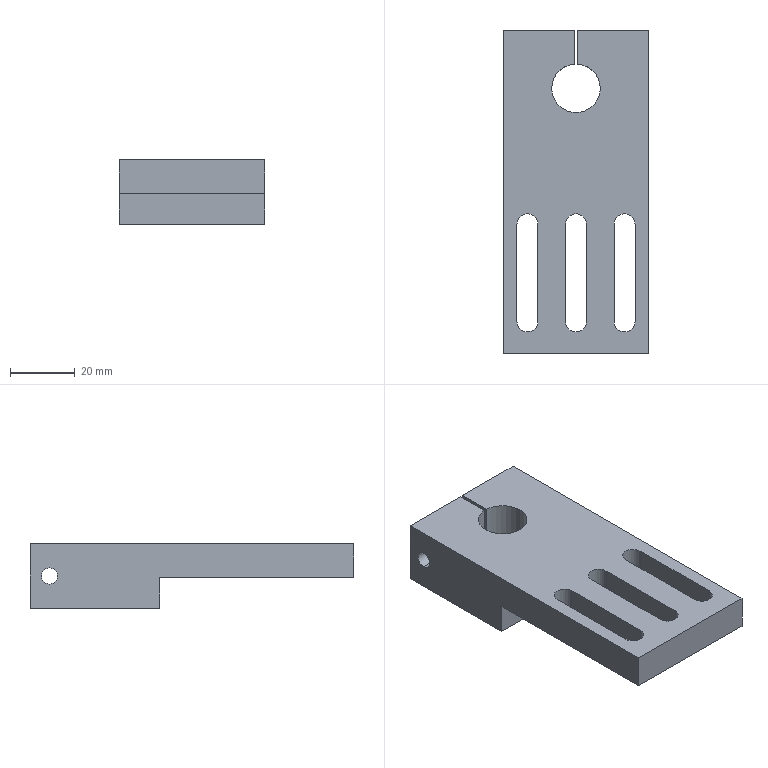Component | SolidWorks | DC-024-24-1 | 1 solid | 33 faces | box 45 x 100 x 20 mm | volume 51844 mm3 | plane 18 | cylinder 15 | commonest cylinder face diameters 6.5 x6 15 x3 5 x2 11 x2 6.6 x2
STEP:
#1=COLOUR_RGB('',0.7922,0.8196,0.9333);
#2=FILL_AREA_STYLE_COLOUR('',#1);
#3=FILL_AREA_STYLE('',(#2));
#4=SURFACE_STYLE_FILL_AREA(#3);
#5=SURFACE_SIDE_STYLE('',(#4));
#6=SURFACE_STYLE_USAGE(.BOTH.,#5);
#7=PRESENTATION_STYLE_ASSIGNMENT((#6));
#8=CARTESIAN_POINT('',(-1.895,12.89,0.6299));
#9=VERTEX_POINT('',#8);
#10=CARTESIAN_POINT('',(-1.895,12.89,0.4331));
#11=VERTEX_POINT('',#10);
#12=CARTESIAN_POINT('',(-1.895,12.89,0.5315));
#13=DIRECTION('',(1.,0.,0.));
#14=DIRECTION('',(0.,0.,-1.));
#15=AXIS2_PLACEMENT_3D('',#12,#13,#14);
#16=CIRCLE('',#15,0.09843);
#17=EDGE_CURVE('',#9,#11,#16,.T.);
#18=ORIENTED_EDGE('',*,*,#17,.F.);
#19=CARTESIAN_POINT('',(-1.029,12.89,0.6299));
#20=VERTEX_POINT('',#19);
#21=CARTESIAN_POINT('',(-1.029,12.89,0.6299));
#22=DIRECTION('',(1.,0.,0.));
#23=VECTOR('',#22,39.37);
#24=LINE('',#21,#23);
#25=EDGE_CURVE('',#9,#20,#24,.T.);
#26=ORIENTED_EDGE('',*,*,#25,.T.);
#27=CARTESIAN_POINT('',(-1.029,12.89,0.4331));
#28=VERTEX_POINT('',#27);
#29=CARTESIAN_POINT('',(-1.029,12.89,0.5315));
#30=DIRECTION('',(1.,0.,0.));
#31=DIRECTION('',(0.,0.,-1.));
#32=AXIS2_PLACEMENT_3D('',#29,#30,#31);
#33=CIRCLE('',#32,0.09843);
#34=EDGE_CURVE('',#20,#28,#33,.T.);
#35=ORIENTED_EDGE('',*,*,#34,.T.);
#36=CARTESIAN_POINT('',(-1.029,12.89,0.4331));
#37=DIRECTION('',(1.,0.,0.));
#38=VECTOR('',#37,39.37);
#39=LINE('',#36,#38);
#40=EDGE_CURVE('',#11,#28,#39,.T.);
#41=ORIENTED_EDGE('',*,*,#40,.F.);
#42=EDGE_LOOP('',(#18,#26,#35,#41));
#43=FACE_OUTER_BOUND('',#42,.T.);
#44=CARTESIAN_POINT('',(-1.029,12.89,0.5315));
#45=DIRECTION('',(1.,0.,0.));
#46=DIRECTION('',(0.,0.,-1.));
#47=AXIS2_PLACEMENT_3D('',#44,#45,#46);
#48=CYLINDRICAL_SURFACE('',#47,0.09843);
#49=ADVANCED_FACE('',(#43),#48,.F.);
#50=CARTESIAN_POINT('',(-0.3753,12.89,0.748));
#51=VERTEX_POINT('',#50);
#52=CARTESIAN_POINT('',(-0.3753,12.89,0.315));
#53=VERTEX_POINT('',#52);
#54=CARTESIAN_POINT('',(-0.3753,12.89,0.5315));
#55=DIRECTION('',(1.,0.,0.));
#56=DIRECTION('',(0.,0.,-1.));
#57=AXIS2_PLACEMENT_3D('',#54,#55,#56);
#58=CIRCLE('',#57,0.2165);
#59=EDGE_CURVE('',#51,#53,#58,.T.);
#60=ORIENTED_EDGE('',*,*,#59,.F.);
#61=CARTESIAN_POINT('',(-0.1233,12.89,0.748));
#62=VERTEX_POINT('',#61);
#63=CARTESIAN_POINT('',(-0.1233,12.89,0.748));
#64=DIRECTION('',(1.,0.,0.));
#65=VECTOR('',#64,39.37);
#66=LINE('',#63,#65);
#67=EDGE_CURVE('',#51,#62,#66,.T.);
#68=ORIENTED_EDGE('',*,*,#67,.T.);
#69=CARTESIAN_POINT('',(-0.1233,12.89,0.315));
#70=VERTEX_POINT('',#69);
#71=CARTESIAN_POINT('',(-0.1233,12.89,0.5315));
#72=DIRECTION('',(1.,0.,0.));
#73=DIRECTION('',(0.,0.,-1.));
#74=AXIS2_PLACEMENT_3D('',#71,#72,#73);
#75=CIRCLE('',#74,0.2165);
#76=EDGE_CURVE('',#62,#70,#75,.T.);
#77=ORIENTED_EDGE('',*,*,#76,.T.);
#78=CARTESIAN_POINT('',(-0.1233,12.89,0.315));
#79=DIRECTION('',(1.,0.,0.));
#80=VECTOR('',#79,39.37);
#81=LINE('',#78,#80);
#82=EDGE_CURVE('',#53,#70,#81,.T.);
#83=ORIENTED_EDGE('',*,*,#82,.F.);
#84=EDGE_LOOP('',(#60,#68,#77,#83));
#85=FACE_OUTER_BOUND('',#84,.T.);
#86=CARTESIAN_POINT('',(-0.1233,12.89,0.5315));
#87=DIRECTION('',(1.,0.,0.));
#88=DIRECTION('',(0.,0.,-1.));
#89=AXIS2_PLACEMENT_3D('',#86,#87,#88);
#90=CYLINDRICAL_SURFACE('',#89,0.2165);
#91=ADVANCED_FACE('',(#85),#90,.F.);
#92=CARTESIAN_POINT('',(-0.9895,12.89,0.6614));
#93=VERTEX_POINT('',#92);
#94=CARTESIAN_POINT('',(-0.9895,12.89,0.4016));
#95=VERTEX_POINT('',#94);
#96=CARTESIAN_POINT('',(-0.9895,12.89,0.5315));
#97=DIRECTION('',(1.,0.,0.));
#98=DIRECTION('',(0.,0.,-1.));
#99=AXIS2_PLACEMENT_3D('',#96,#97,#98);
#100=CIRCLE('',#99,0.1299);
#101=EDGE_CURVE('',#93,#95,#100,.T.);
#102=ORIENTED_EDGE('',*,*,#101,.F.);
#103=CARTESIAN_POINT('',(-0.3753,12.89,0.6614));
#104=VERTEX_POINT('',#103);
#105=CARTESIAN_POINT('',(-0.1233,12.89,0.6614));
#106=DIRECTION('',(1.,0.,0.));
#107=VECTOR('',#106,39.37);
#108=LINE('',#105,#107);
#109=EDGE_CURVE('',#93,#104,#108,.T.);
#110=ORIENTED_EDGE('',*,*,#109,.T.);
#111=CARTESIAN_POINT('',(-0.3753,12.89,0.4016));
#112=VERTEX_POINT('',#111);
#113=CARTESIAN_POINT('',(-0.3753,12.89,0.5315));
#114=DIRECTION('',(1.,0.,0.));
#115=DIRECTION('',(0.,0.,-1.));
#116=AXIS2_PLACEMENT_3D('',#113,#114,#115);
#117=CIRCLE('',#116,0.1299);
#118=EDGE_CURVE('',#104,#112,#117,.T.);
#119=ORIENTED_EDGE('',*,*,#118,.T.);
#120=CARTESIAN_POINT('',(-0.1233,12.89,0.4016));
#121=DIRECTION('',(1.,0.,0.));
#122=VECTOR('',#121,39.37);
#123=LINE('',#120,#122);
#124=EDGE_CURVE('',#95,#112,#123,.T.);
#125=ORIENTED_EDGE('',*,*,#124,.F.);
#126=EDGE_LOOP('',(#102,#110,#119,#125));
#127=FACE_OUTER_BOUND('',#126,.T.);
#128=CARTESIAN_POINT('',(-0.1233,12.89,0.5315));
#129=DIRECTION('',(1.,0.,0.));
#130=DIRECTION('',(0.,0.,-1.));
#131=AXIS2_PLACEMENT_3D('',#128,#129,#130);
#132=CYLINDRICAL_SURFACE('',#131,0.1299);
#133=ADVANCED_FACE('',(#127),#132,.F.);
#134=CARTESIAN_POINT('',(-0.7139,12.418,0.1378));
#135=VERTEX_POINT('',#134);
#136=CARTESIAN_POINT('',(-1.304,12.418,0.1378));
#137=VERTEX_POINT('',#136);
#138=CARTESIAN_POINT('',(-1.009,12.418,0.1378));
#139=DIRECTION('',(0.,0.,-1.));
#140=DIRECTION('',(1.,0.,0.));
#141=AXIS2_PLACEMENT_3D('',#138,#139,#140);
#142=CIRCLE('',#141,0.2953);
#143=EDGE_CURVE('',#135,#137,#142,.T.);
#144=ORIENTED_EDGE('',*,*,#143,.T.);
#145=CARTESIAN_POINT('',(-1.304,12.418,0.9252));
#146=VERTEX_POINT('',#145);
#147=CARTESIAN_POINT('',(-1.304,12.418,-0.6974));
#148=DIRECTION('',(0.,0.,1.));
#149=VECTOR('',#148,39.37);
#150=LINE('',#147,#149);
#151=EDGE_CURVE('',#137,#146,#150,.T.);
#152=ORIENTED_EDGE('',*,*,#151,.T.);
#153=CARTESIAN_POINT('',(-0.7139,12.418,0.9252));
#154=VERTEX_POINT('',#153);
#155=CARTESIAN_POINT('',(-1.009,12.418,0.9252));
#156=DIRECTION('',(0.,0.,1.));
#157=DIRECTION('',(1.,0.,0.));
#158=AXIS2_PLACEMENT_3D('',#155,#156,#157);
#159=CIRCLE('',#158,0.2953);
#160=EDGE_CURVE('',#146,#154,#159,.T.);
#161=ORIENTED_EDGE('',*,*,#160,.T.);
#162=CARTESIAN_POINT('',(-0.7139,12.418,-0.6974));
#163=DIRECTION('',(0.,0.,1.));
#164=VECTOR('',#163,39.37);
#165=LINE('',#162,#164);
#166=EDGE_CURVE('',#135,#154,#165,.T.);
#167=ORIENTED_EDGE('',*,*,#166,.F.);
#168=EDGE_LOOP('',(#144,#152,#161,#167));
#169=FACE_OUTER_BOUND('',#168,.T.);
#170=CARTESIAN_POINT('',(-1.009,12.418,-0.6974));
#171=DIRECTION('',(0.,0.,1.));
#172=DIRECTION('',(1.,0.,0.));
#173=AXIS2_PLACEMENT_3D('',#170,#171,#172);
#174=CYLINDRICAL_SURFACE('',#173,0.2953);
#175=ADVANCED_FACE('',(#169),#174,.F.);
#176=CARTESIAN_POINT('',(-0.9895,12.712,0.1378));
#177=VERTEX_POINT('',#176);
#178=CARTESIAN_POINT('',(-1.009,12.418,0.1378));
#179=DIRECTION('',(0.,0.,-1.));
#180=DIRECTION('',(1.,0.,0.));
#181=AXIS2_PLACEMENT_3D('',#178,#179,#180);
#182=CIRCLE('',#181,0.2953);
#183=EDGE_CURVE('',#177,#135,#182,.T.);
#184=ORIENTED_EDGE('',*,*,#183,.T.);
#185=ORIENTED_EDGE('',*,*,#166,.T.);
#186=CARTESIAN_POINT('',(-0.9895,12.712,0.9252));
#187=VERTEX_POINT('',#186);
#188=CARTESIAN_POINT('',(-1.009,12.418,0.9252));
#189=DIRECTION('',(0.,0.,1.));
#190=DIRECTION('',(1.,0.,0.));
#191=AXIS2_PLACEMENT_3D('',#188,#189,#190);
#192=CIRCLE('',#191,0.2953);
#193=EDGE_CURVE('',#154,#187,#192,.T.);
#194=ORIENTED_EDGE('',*,*,#193,.T.);
#195=CARTESIAN_POINT('',(-0.9895,12.712,-0.6974));
#196=DIRECTION('',(0.,0.,-1.));
#197=VECTOR('',#196,39.37);
#198=LINE('',#195,#197);
#199=EDGE_CURVE('',#187,#177,#198,.T.);
#200=ORIENTED_EDGE('',*,*,#199,.T.);
#201=EDGE_LOOP('',(#184,#185,#194,#200));
#202=FACE_OUTER_BOUND('',#201,.T.);
#203=CARTESIAN_POINT('',(-1.009,12.418,-0.6974));
#204=DIRECTION('',(0.,0.,1.));
#205=DIRECTION('',(1.,0.,0.));
#206=AXIS2_PLACEMENT_3D('',#203,#204,#205);
#207=CYLINDRICAL_SURFACE('',#206,0.2953);
#208=ADVANCED_FACE('',(#202),#207,.F.);
#209=CARTESIAN_POINT('',(-0.1233,9.189,0.9252));
#210=VERTEX_POINT('',#209);
#211=CARTESIAN_POINT('',(-0.1233,9.189,0.5118));
#212=VERTEX_POINT('',#211);
#213=CARTESIAN_POINT('',(-0.1233,9.189,0.9252));
#214=DIRECTION('',(0.,0.,-1.));
#215=VECTOR('',#214,39.37);
#216=LINE('',#213,#215);
#217=EDGE_CURVE('',#210,#212,#216,.T.);
#218=ORIENTED_EDGE('',*,*,#217,.T.);
#219=CARTESIAN_POINT('',(-0.1233,11.552,0.5118));
#220=VERTEX_POINT('',#219);
#221=CARTESIAN_POINT('',(-0.1233,9.189,0.5118));
#222=DIRECTION('',(0.,-1.,0.));
#223=VECTOR('',#222,39.37);
#224=LINE('',#221,#223);
#225=EDGE_CURVE('',#220,#212,#224,.T.);
#226=ORIENTED_EDGE('',*,*,#225,.F.);
#227=CARTESIAN_POINT('',(-0.1233,11.552,0.1378));
#228=VERTEX_POINT('',#227);
#229=CARTESIAN_POINT('',(-0.1233,11.552,0.1378));
#230=DIRECTION('',(0.,-0.,1.));
#231=VECTOR('',#230,39.37);
#232=LINE('',#229,#231);
#233=EDGE_CURVE('',#228,#220,#232,.T.);
#234=ORIENTED_EDGE('',*,*,#233,.F.);
#235=CARTESIAN_POINT('',(-0.1233,13.126,0.1378));
#236=VERTEX_POINT('',#235);
#237=CARTESIAN_POINT('',(-0.1233,9.189,0.1378));
#238=DIRECTION('',(0.,1.,0.));
#239=VECTOR('',#238,39.37);
#240=LINE('',#237,#239);
#241=EDGE_CURVE('',#228,#236,#240,.T.);
#242=ORIENTED_EDGE('',*,*,#241,.T.);
#243=CARTESIAN_POINT('',(-0.1233,13.126,0.9252));
#244=VERTEX_POINT('',#243);
#245=CARTESIAN_POINT('',(-0.1233,13.126,0.9252));
#246=DIRECTION('',(0.,0.,-1.));
#247=VECTOR('',#246,39.37);
#248=LINE('',#245,#247);
#249=EDGE_CURVE('',#244,#236,#248,.T.);
#250=ORIENTED_EDGE('',*,*,#249,.F.);
#251=CARTESIAN_POINT('',(-0.1233,9.189,0.9252));
#252=DIRECTION('',(0.,1.,0.));
#253=VECTOR('',#252,39.37);
#254=LINE('',#251,#253);
#255=EDGE_CURVE('',#210,#244,#254,.T.);
#256=ORIENTED_EDGE('',*,*,#255,.F.);
#257=EDGE_LOOP('',(#218,#226,#234,#242,#250,#256));
#258=FACE_OUTER_BOUND('',#257,.T.);
#259=CARTESIAN_POINT('',(-0.1233,12.89,0.5315));
#260=DIRECTION('',(1.,0.,0.));
#261=DIRECTION('',(0.,0.,-1.));
#262=AXIS2_PLACEMENT_3D('',#259,#260,#261);
#263=CIRCLE('',#262,0.2165);
#264=EDGE_CURVE('',#70,#62,#263,.T.);
#265=ORIENTED_EDGE('',*,*,#264,.F.);
#266=ORIENTED_EDGE('',*,*,#76,.F.);
#267=EDGE_LOOP('',(#265,#266));
#268=FACE_BOUND('',#267,.T.);
#269=CARTESIAN_POINT('',(-0.1233,9.189,0.9252));
#270=DIRECTION('',(-1.,0.,0.));
#271=DIRECTION('',(0.,0.,1.));
#272=AXIS2_PLACEMENT_3D('',#269,#270,#271);
#273=PLANE('',#272);
#274=ADVANCED_FACE('',(#258,#268),#273,.F.);
#275=CARTESIAN_POINT('',(-1.029,13.126,0.9252));
#276=VERTEX_POINT('',#275);
#277=CARTESIAN_POINT('',(-1.895,13.126,0.9252));
#278=VERTEX_POINT('',#277);
#279=CARTESIAN_POINT('',(-0.1233,13.126,0.9252));
#280=DIRECTION('',(-1.,-0.,0.));
#281=VECTOR('',#280,39.37);
#282=LINE('',#279,#281);
#283=EDGE_CURVE('',#276,#278,#282,.T.);
#284=ORIENTED_EDGE('',*,*,#283,.F.);
#285=CARTESIAN_POINT('',(-1.029,13.126,0.1378));
#286=VERTEX_POINT('',#285);
#287=CARTESIAN_POINT('',(-1.029,13.126,0.9252));
#288=DIRECTION('',(0.,0.,-1.));
#289=VECTOR('',#288,39.37);
#290=LINE('',#287,#289);
#291=EDGE_CURVE('',#276,#286,#290,.T.);
#292=ORIENTED_EDGE('',*,*,#291,.T.);
#293=CARTESIAN_POINT('',(-1.895,13.126,0.1378));
#294=VERTEX_POINT('',#293);
#295=CARTESIAN_POINT('',(-0.1233,13.126,0.1378));
#296=DIRECTION('',(-1.,-0.,0.));
#297=VECTOR('',#296,39.37);
#298=LINE('',#295,#297);
#299=EDGE_CURVE('',#286,#294,#298,.T.);
#300=ORIENTED_EDGE('',*,*,#299,.T.);
#301=CARTESIAN_POINT('',(-1.895,13.126,0.9252));
#302=DIRECTION('',(0.,0.,-1.));
#303=VECTOR('',#302,39.37);
#304=LINE('',#301,#303);
#305=EDGE_CURVE('',#278,#294,#304,.T.);
#306=ORIENTED_EDGE('',*,*,#305,.F.);
#307=EDGE_LOOP('',(#284,#292,#300,#306));
#308=FACE_OUTER_BOUND('',#307,.T.);
#309=CARTESIAN_POINT('',(-0.1233,13.126,0.9252));
#310=DIRECTION('',(0.,-1.,0.));
#311=DIRECTION('',(1.,0.,0.));
#312=AXIS2_PLACEMENT_3D('',#309,#310,#311);
#313=PLANE('',#312);
#314=ADVANCED_FACE('',(#308),#313,.F.);
#315=CARTESIAN_POINT('',(-1.895,12.89,0.5315));
#316=DIRECTION('',(1.,0.,0.));
#317=DIRECTION('',(0.,0.,-1.));
#318=AXIS2_PLACEMENT_3D('',#315,#316,#317);
#319=CIRCLE('',#318,0.09843);
#320=EDGE_CURVE('',#11,#9,#319,.T.);
#321=ORIENTED_EDGE('',*,*,#320,.T.);
#322=ORIENTED_EDGE('',*,*,#17,.T.);
#323=EDGE_LOOP('',(#321,#322));
#324=FACE_BOUND('',#323,.T.);
#325=CARTESIAN_POINT('',(-1.895,11.552,0.5118));
#326=VERTEX_POINT('',#325);
#327=CARTESIAN_POINT('',(-1.895,11.552,0.1378));
#328=VERTEX_POINT('',#327);
#329=CARTESIAN_POINT('',(-1.895,11.552,0.1378));
#330=DIRECTION('',(0.,0.,-1.));
#331=VECTOR('',#330,39.37);
#332=LINE('',#329,#331);
#333=EDGE_CURVE('',#326,#328,#332,.T.);
#334=ORIENTED_EDGE('',*,*,#333,.F.);
#335=CARTESIAN_POINT('',(-1.895,9.189,0.5118));
#336=VERTEX_POINT('',#335);
#337=CARTESIAN_POINT('',(-1.895,9.189,0.5118));
#338=DIRECTION('',(0.,1.,0.));
#339=VECTOR('',#338,39.37);
#340=LINE('',#337,#339);
#341=EDGE_CURVE('',#336,#326,#340,.T.);
#342=ORIENTED_EDGE('',*,*,#341,.F.);
#343=CARTESIAN_POINT('',(-1.895,9.189,0.9252));
#344=VERTEX_POINT('',#343);
#345=CARTESIAN_POINT('',(-1.895,9.189,0.9252));
#346=DIRECTION('',(0.,0.,-1.));
#347=VECTOR('',#346,39.37);
#348=LINE('',#345,#347);
#349=EDGE_CURVE('',#344,#336,#348,.T.);
#350=ORIENTED_EDGE('',*,*,#349,.F.);
#351=CARTESIAN_POINT('',(-1.895,9.189,0.9252));
#352=DIRECTION('',(0.,-1.,0.));
#353=VECTOR('',#352,39.37);
#354=LINE('',#351,#353);
#355=EDGE_CURVE('',#278,#344,#354,.T.);
#356=ORIENTED_EDGE('',*,*,#355,.F.);
#357=ORIENTED_EDGE('',*,*,#305,.T.);
#358=CARTESIAN_POINT('',(-1.895,9.189,0.1378));
#359=DIRECTION('',(0.,-1.,0.));
#360=VECTOR('',#359,39.37);
#361=LINE('',#358,#360);
#362=EDGE_CURVE('',#294,#328,#361,.T.);
#363=ORIENTED_EDGE('',*,*,#362,.T.);
#364=EDGE_LOOP('',(#334,#342,#350,#356,#357,#363));
#365=FACE_OUTER_BOUND('',#364,.T.);
#366=CARTESIAN_POINT('',(-1.895,9.189,0.9252));
#367=DIRECTION('',(1.,0.,0.));
#368=DIRECTION('',(0.,0.,-1.));
#369=AXIS2_PLACEMENT_3D('',#366,#367,#368);
#370=PLANE('',#369);
#371=ADVANCED_FACE('',(#324,#365),#370,.F.);
#372=ORIENTED_EDGE('',*,*,#349,.T.);
#373=CARTESIAN_POINT('',(-4.287,9.189,0.5118));
#374=DIRECTION('',(1.,0.,0.));
#375=VECTOR('',#374,39.37);
#376=LINE('',#373,#375);
#377=EDGE_CURVE('',#336,#212,#376,.T.);
#378=ORIENTED_EDGE('',*,*,#377,.T.);
#379=ORIENTED_EDGE('',*,*,#217,.F.);
#380=CARTESIAN_POINT('',(-0.1233,9.189,0.9252));
#381=DIRECTION('',(1.,0.,0.));
#382=VECTOR('',#381,39.37);
#383=LINE('',#380,#382);
#384=EDGE_CURVE('',#344,#210,#383,.T.);
#385=ORIENTED_EDGE('',*,*,#384,.F.);
#386=EDGE_LOOP('',(#372,#378,#379,#385));
#387=FACE_OUTER_BOUND('',#386,.T.);
#388=CARTESIAN_POINT('',(-0.1233,9.189,0.9252));
#389=DIRECTION('',(-0.,1.,0.));
#390=DIRECTION('',(-1.,-0.,0.));
#391=AXIS2_PLACEMENT_3D('',#388,#389,#390);
#392=PLANE('',#391);
#393=ADVANCED_FACE('',(#387),#392,.F.);
#394=CARTESIAN_POINT('',(-0.9895,13.126,0.1378));
#395=VERTEX_POINT('',#394);
#396=CARTESIAN_POINT('',(-0.1233,13.126,0.1378));
#397=DIRECTION('',(-1.,-0.,0.));
#398=VECTOR('',#397,39.37);
#399=LINE('',#396,#398);
#400=EDGE_CURVE('',#236,#395,#399,.T.);
#401=ORIENTED_EDGE('',*,*,#400,.T.);
#402=CARTESIAN_POINT('',(-0.9895,13.126,0.9252));
#403=VERTEX_POINT('',#402);
#404=CARTESIAN_POINT('',(-0.9895,13.126,0.9252));
#405=DIRECTION('',(0.,0.,1.));
#406=VECTOR('',#405,39.37);
#407=LINE('',#404,#406);
#408=EDGE_CURVE('',#395,#403,#407,.T.);
#409=ORIENTED_EDGE('',*,*,#408,.T.);
#410=CARTESIAN_POINT('',(-0.1233,13.126,0.9252));
#411=DIRECTION('',(-1.,-0.,0.));
#412=VECTOR('',#411,39.37);
#413=LINE('',#410,#412);
#414=EDGE_CURVE('',#244,#403,#413,.T.);
#415=ORIENTED_EDGE('',*,*,#414,.F.);
#416=ORIENTED_EDGE('',*,*,#249,.T.);
#417=EDGE_LOOP('',(#401,#409,#415,#416));
#418=FACE_OUTER_BOUND('',#417,.T.);
#419=CARTESIAN_POINT('',(-0.1233,13.126,0.9252));
#420=DIRECTION('',(0.,-1.,0.));
#421=DIRECTION('',(1.,0.,0.));
#422=AXIS2_PLACEMENT_3D('',#419,#420,#421);
#423=PLANE('',#422);
#424=ADVANCED_FACE('',(#418),#423,.F.);
#425=CARTESIAN_POINT('',(-1.472,10.764,0.9252));
#426=VERTEX_POINT('',#425);
#427=CARTESIAN_POINT('',(-1.728,10.764,0.9252));
#428=VERTEX_POINT('',#427);
#429=CARTESIAN_POINT('',(-1.6,10.764,0.9252));
#430=DIRECTION('',(0.,0.,1.));
#431=DIRECTION('',(1.,0.,0.));
#432=AXIS2_PLACEMENT_3D('',#429,#430,#431);
#433=CIRCLE('',#432,0.128);
#434=EDGE_CURVE('',#426,#428,#433,.T.);
#435=ORIENTED_EDGE('',*,*,#434,.F.);
#436=CARTESIAN_POINT('',(-1.472,9.583,0.9252));
#437=VERTEX_POINT('',#436);
#438=CARTESIAN_POINT('',(-1.472,10.764,0.9252));
#439=DIRECTION('',(-0.,1.,0.));
#440=VECTOR('',#439,39.37);
#441=LINE('',#438,#440);
#442=EDGE_CURVE('',#437,#426,#441,.T.);
#443=ORIENTED_EDGE('',*,*,#442,.F.);
#444=CARTESIAN_POINT('',(-1.728,9.583,0.9252));
#445=VERTEX_POINT('',#444);
#446=CARTESIAN_POINT('',(-1.6,9.583,0.9252));
#447=DIRECTION('',(0.,0.,1.));
#448=DIRECTION('',(1.,0.,0.));
#449=AXIS2_PLACEMENT_3D('',#446,#447,#448);
#450=CIRCLE('',#449,0.128);
#451=EDGE_CURVE('',#445,#437,#450,.T.);
#452=ORIENTED_EDGE('',*,*,#451,.F.);
#453=CARTESIAN_POINT('',(-1.728,10.764,0.9252));
#454=DIRECTION('',(0.,-1.,0.));
#455=VECTOR('',#454,39.37);
#456=LINE('',#453,#455);
#457=EDGE_CURVE('',#428,#445,#456,.T.);
#458=ORIENTED_EDGE('',*,*,#457,.F.);
#459=EDGE_LOOP('',(#435,#443,#452,#458));
#460=FACE_BOUND('',#459,.T.);
#461=CARTESIAN_POINT('',(-0.2907,10.764,0.9252));
#462=VERTEX_POINT('',#461);
#463=CARTESIAN_POINT('',(-0.5466,10.764,0.9252));
#464=VERTEX_POINT('',#463);
#465=CARTESIAN_POINT('',(-0.4186,10.764,0.9252));
#466=DIRECTION('',(0.,0.,1.));
#467=DIRECTION('',(1.,0.,0.));
#468=AXIS2_PLACEMENT_3D('',#465,#466,#467);
#469=CIRCLE('',#468,0.128);
#470=EDGE_CURVE('',#462,#464,#469,.T.);
#471=ORIENTED_EDGE('',*,*,#470,.F.);
#472=CARTESIAN_POINT('',(-0.2907,9.583,0.9252));
#473=VERTEX_POINT('',#472);
#474=CARTESIAN_POINT('',(-0.2907,10.764,0.9252));
#475=DIRECTION('',(-0.,1.,0.));
#476=VECTOR('',#475,39.37);
#477=LINE('',#474,#476);
#478=EDGE_CURVE('',#473,#462,#477,.T.);
#479=ORIENTED_EDGE('',*,*,#478,.F.);
#480=CARTESIAN_POINT('',(-0.5466,9.583,0.9252));
#481=VERTEX_POINT('',#480);
#482=CARTESIAN_POINT('',(-0.4186,9.583,0.9252));
#483=DIRECTION('',(0.,0.,1.));
#484=DIRECTION('',(1.,0.,0.));
#485=AXIS2_PLACEMENT_3D('',#482,#483,#484);
#486=CIRCLE('',#485,0.128);
#487=EDGE_CURVE('',#481,#473,#486,.T.);
#488=ORIENTED_EDGE('',*,*,#487,.F.);
#489=CARTESIAN_POINT('',(-0.5466,10.764,0.9252));
#490=DIRECTION('',(0.,-1.,0.));
#491=VECTOR('',#490,39.37);
#492=LINE('',#489,#491);
#493=EDGE_CURVE('',#464,#481,#492,.T.);
#494=ORIENTED_EDGE('',*,*,#493,.F.);
#495=EDGE_LOOP('',(#471,#479,#488,#494));
#496=FACE_BOUND('',#495,.T.);
#497=CARTESIAN_POINT('',(-0.8812,10.764,0.9252));
#498=VERTEX_POINT('',#497);
#499=CARTESIAN_POINT('',(-1.137,10.764,0.9252));
#500=VERTEX_POINT('',#499);
#501=CARTESIAN_POINT('',(-1.009,10.764,0.9252));
#502=DIRECTION('',(0.,0.,1.));
#503=DIRECTION('',(1.,0.,0.));
#504=AXIS2_PLACEMENT_3D('',#501,#502,#503);
#505=CIRCLE('',#504,0.128);
#506=EDGE_CURVE('',#498,#500,#505,.T.);
#507=ORIENTED_EDGE('',*,*,#506,.F.);
#508=CARTESIAN_POINT('',(-0.8812,9.583,0.9252));
#509=VERTEX_POINT('',#508);
#510=CARTESIAN_POINT('',(-0.8812,10.764,0.9252));
#511=DIRECTION('',(-0.,1.,0.));
#512=VECTOR('',#511,39.37);
#513=LINE('',#510,#512);
#514=EDGE_CURVE('',#509,#498,#513,.T.);
#515=ORIENTED_EDGE('',*,*,#514,.F.);
#516=CARTESIAN_POINT('',(-1.137,9.583,0.9252));
#517=VERTEX_POINT('',#516);
#518=CARTESIAN_POINT('',(-1.009,9.583,0.9252));
#519=DIRECTION('',(0.,0.,1.));
#520=DIRECTION('',(1.,0.,0.));
#521=AXIS2_PLACEMENT_3D('',#518,#519,#520);
#522=CIRCLE('',#521,0.128);
#523=EDGE_CURVE('',#517,#509,#522,.T.);
#524=ORIENTED_EDGE('',*,*,#523,.F.);
#525=CARTESIAN_POINT('',(-1.137,10.764,0.9252));
#526=DIRECTION('',(0.,-1.,0.));
#527=VECTOR('',#526,39.37);
#528=LINE('',#525,#527);
#529=EDGE_CURVE('',#500,#517,#528,.T.);
#530=ORIENTED_EDGE('',*,*,#529,.F.);
#531=EDGE_LOOP('',(#507,#515,#524,#530));
#532=FACE_BOUND('',#531,.T.);
#533=CARTESIAN_POINT('',(-1.029,12.712,0.9252));
#534=VERTEX_POINT('',#533);
#535=CARTESIAN_POINT('',(-1.029,14.13,0.9252));
#536=DIRECTION('',(0.,-1.,0.));
#537=VECTOR('',#536,39.37);
#538=LINE('',#535,#537);
#539=EDGE_CURVE('',#276,#534,#538,.T.);
#540=ORIENTED_EDGE('',*,*,#539,.F.);
#541=ORIENTED_EDGE('',*,*,#283,.T.);
#542=ORIENTED_EDGE('',*,*,#355,.T.);
#543=ORIENTED_EDGE('',*,*,#384,.T.);
#544=ORIENTED_EDGE('',*,*,#255,.T.);
#545=ORIENTED_EDGE('',*,*,#414,.T.);
#546=CARTESIAN_POINT('',(-0.9895,14.13,0.9252));
#547=DIRECTION('',(0.,1.,0.));
#548=VECTOR('',#547,39.37);
#549=LINE('',#546,#548);
#550=EDGE_CURVE('',#187,#403,#549,.T.);
#551=ORIENTED_EDGE('',*,*,#550,.F.);
#552=ORIENTED_EDGE('',*,*,#193,.F.);
#553=ORIENTED_EDGE('',*,*,#160,.F.);
#554=CARTESIAN_POINT('',(-1.009,12.418,0.9252));
#555=DIRECTION('',(0.,0.,1.));
#556=DIRECTION('',(1.,0.,0.));
#557=AXIS2_PLACEMENT_3D('',#554,#555,#556);
#558=CIRCLE('',#557,0.2953);
#559=EDGE_CURVE('',#534,#146,#558,.T.);
#560=ORIENTED_EDGE('',*,*,#559,.F.);
#561=EDGE_LOOP('',(#540,#541,#542,#543,#544,#545,#551,#552,#553,#560));
#562=FACE_OUTER_BOUND('',#561,.T.);
#563=CARTESIAN_POINT('',(-1.009,11.158,0.9252));
#564=DIRECTION('',(0.,0.,1.));
#565=DIRECTION('',(1.,0.,0.));
#566=AXIS2_PLACEMENT_3D('',#563,#564,#565);
#567=PLANE('',#566);
#568=ADVANCED_FACE('',(#460,#496,#532,#562),#567,.T.);
#569=ORIENTED_EDGE('',*,*,#241,.F.);
#570=CARTESIAN_POINT('',(-4.287,11.552,0.1378));
#571=DIRECTION('',(1.,0.,0.));
#572=VECTOR('',#571,39.37);
#573=LINE('',#570,#572);
#574=EDGE_CURVE('',#328,#228,#573,.T.);
#575=ORIENTED_EDGE('',*,*,#574,.F.);
#576=ORIENTED_EDGE('',*,*,#362,.F.);
#577=ORIENTED_EDGE('',*,*,#299,.F.);
#578=CARTESIAN_POINT('',(-1.029,12.712,0.1378));
#579=VERTEX_POINT('',#578);
#580=CARTESIAN_POINT('',(-1.029,14.13,0.1378));
#581=DIRECTION('',(0.,1.,0.));
#582=VECTOR('',#581,39.37);
#583=LINE('',#580,#582);
#584=EDGE_CURVE('',#579,#286,#583,.T.);
#585=ORIENTED_EDGE('',*,*,#584,.F.);
#586=CARTESIAN_POINT('',(-1.009,12.418,0.1378));
#587=DIRECTION('',(0.,0.,-1.));
#588=DIRECTION('',(1.,0.,0.));
#589=AXIS2_PLACEMENT_3D('',#586,#587,#588);
#590=CIRCLE('',#589,0.2953);
#591=EDGE_CURVE('',#137,#579,#590,.T.);
#592=ORIENTED_EDGE('',*,*,#591,.F.);
#593=ORIENTED_EDGE('',*,*,#143,.F.);
#594=ORIENTED_EDGE('',*,*,#183,.F.);
#595=CARTESIAN_POINT('',(-0.9895,14.13,0.1378));
#596=DIRECTION('',(0.,-1.,0.));
#597=VECTOR('',#596,39.37);
#598=LINE('',#595,#597);
#599=EDGE_CURVE('',#395,#177,#598,.T.);
#600=ORIENTED_EDGE('',*,*,#599,.F.);
#601=ORIENTED_EDGE('',*,*,#400,.F.);
#602=EDGE_LOOP('',(#569,#575,#576,#577,#585,#592,#593,#594,#600,#601));
#603=FACE_OUTER_BOUND('',#602,.T.);
#604=CARTESIAN_POINT('',(-1.009,11.158,0.1378));
#605=DIRECTION('',(0.,0.,1.));
#606=DIRECTION('',(1.,0.,0.));
#607=AXIS2_PLACEMENT_3D('',#604,#605,#606);
#608=PLANE('',#607);
#609=ADVANCED_FACE('',(#603),#608,.F.);
#610=ORIENTED_EDGE('',*,*,#151,.F.);
#611=ORIENTED_EDGE('',*,*,#591,.T.);
#612=CARTESIAN_POINT('',(-1.029,12.712,-0.6974));
#613=DIRECTION('',(0.,0.,1.));
#614=VECTOR('',#613,39.37);
#615=LINE('',#612,#614);
#616=EDGE_CURVE('',#579,#534,#615,.T.);
#617=ORIENTED_EDGE('',*,*,#616,.T.);
#618=ORIENTED_EDGE('',*,*,#559,.T.);
#619=EDGE_LOOP('',(#610,#611,#617,#618));
#620=FACE_OUTER_BOUND('',#619,.T.);
#621=CARTESIAN_POINT('',(-1.009,12.418,-0.6974));
#622=DIRECTION('',(0.,0.,1.));
#623=DIRECTION('',(1.,0.,0.));
#624=AXIS2_PLACEMENT_3D('',#621,#622,#623);
#625=CYLINDRICAL_SURFACE('',#624,0.2953);
#626=ADVANCED_FACE('',(#620),#625,.F.);
#627=CARTESIAN_POINT('',(-0.9895,12.89,0.5315));
#628=DIRECTION('',(1.,0.,0.));
#629=DIRECTION('',(0.,0.,-1.));
#630=AXIS2_PLACEMENT_3D('',#627,#628,#629);
#631=CIRCLE('',#630,0.1299);
#632=EDGE_CURVE('',#95,#93,#631,.T.);
#633=ORIENTED_EDGE('',*,*,#632,.T.);
#634=ORIENTED_EDGE('',*,*,#101,.T.);
#635=EDGE_LOOP('',(#633,#634));
#636=FACE_BOUND('',#635,.T.);
#637=ORIENTED_EDGE('',*,*,#599,.T.);
#638=ORIENTED_EDGE('',*,*,#199,.F.);
#639=ORIENTED_EDGE('',*,*,#550,.T.);
#640=ORIENTED_EDGE('',*,*,#408,.F.);
#641=EDGE_LOOP('',(#637,#638,#639,#640));
#642=FACE_OUTER_BOUND('',#641,.T.);
#643=CARTESIAN_POINT('',(-0.9895,14.13,-1.869));
#644=DIRECTION('',(1.,0.,0.));
#645=DIRECTION('',(0.,0.,-1.));
#646=AXIS2_PLACEMENT_3D('',#643,#644,#645);
#647=PLANE('',#646);
#648=ADVANCED_FACE('',(#636,#642),#647,.F.);
#649=CARTESIAN_POINT('',(-1.029,12.89,0.5315));
#650=DIRECTION('',(1.,0.,0.));
#651=DIRECTION('',(0.,0.,-1.));
#652=AXIS2_PLACEMENT_3D('',#649,#650,#651);
#653=CIRCLE('',#652,0.09843);
#654=EDGE_CURVE('',#28,#20,#653,.T.);
#655=ORIENTED_EDGE('',*,*,#654,.F.);
#656=ORIENTED_EDGE('',*,*,#34,.F.);
#657=EDGE_LOOP('',(#655,#656));
#658=FACE_BOUND('',#657,.T.);
#659=ORIENTED_EDGE('',*,*,#539,.T.);
#660=ORIENTED_EDGE('',*,*,#616,.F.);
#661=ORIENTED_EDGE('',*,*,#584,.T.);
#662=ORIENTED_EDGE('',*,*,#291,.F.);
#663=EDGE_LOOP('',(#659,#660,#661,#662));
#664=FACE_OUTER_BOUND('',#663,.T.);
#665=CARTESIAN_POINT('',(-1.029,14.13,-1.869));
#666=DIRECTION('',(-1.,0.,0.));
#667=DIRECTION('',(0.,0.,1.));
#668=AXIS2_PLACEMENT_3D('',#665,#666,#667);
#669=PLANE('',#668);
#670=ADVANCED_FACE('',(#658,#664),#669,.F.);
#671=ORIENTED_EDGE('',*,*,#109,.F.);
#672=ORIENTED_EDGE('',*,*,#632,.F.);
#673=ORIENTED_EDGE('',*,*,#124,.T.);
#674=CARTESIAN_POINT('',(-0.3753,12.89,0.5315));
#675=DIRECTION('',(1.,0.,0.));
#676=DIRECTION('',(0.,0.,-1.));
#677=AXIS2_PLACEMENT_3D('',#674,#675,#676);
#678=CIRCLE('',#677,0.1299);
#679=EDGE_CURVE('',#112,#104,#678,.T.);
#680=ORIENTED_EDGE('',*,*,#679,.T.);
#681=EDGE_LOOP('',(#671,#672,#673,#680));
#682=FACE_OUTER_BOUND('',#681,.T.);
#683=CARTESIAN_POINT('',(-0.1233,12.89,0.5315));
#684=DIRECTION('',(1.,0.,0.));
#685=DIRECTION('',(0.,0.,-1.));
#686=AXIS2_PLACEMENT_3D('',#683,#684,#685);
#687=CYLINDRICAL_SURFACE('',#686,0.1299);
#688=ADVANCED_FACE('',(#682),#687,.F.);
#689=ORIENTED_EDGE('',*,*,#679,.F.);
#690=ORIENTED_EDGE('',*,*,#118,.F.);
#691=EDGE_LOOP('',(#689,#690));
#692=FACE_BOUND('',#691,.T.);
#693=CARTESIAN_POINT('',(-0.3753,12.89,0.5315));
#694=DIRECTION('',(1.,0.,0.));
#695=DIRECTION('',(0.,0.,-1.));
#696=AXIS2_PLACEMENT_3D('',#693,#694,#695);
#697=CIRCLE('',#696,0.2165);
#698=EDGE_CURVE('',#53,#51,#697,.T.);
#699=ORIENTED_EDGE('',*,*,#698,.T.);
#700=ORIENTED_EDGE('',*,*,#59,.T.);
#701=EDGE_LOOP('',(#699,#700));
#702=FACE_OUTER_BOUND('',#701,.T.);
#703=CARTESIAN_POINT('',(-0.3753,13.02,0.5315));
#704=DIRECTION('',(-1.,0.,0.));
#705=DIRECTION('',(0.,0.,1.));
#706=AXIS2_PLACEMENT_3D('',#703,#704,#705);
#707=PLANE('',#706);
#708=ADVANCED_FACE('',(#692,#702),#707,.F.);
#709=ORIENTED_EDGE('',*,*,#67,.F.);
#710=ORIENTED_EDGE('',*,*,#698,.F.);
#711=ORIENTED_EDGE('',*,*,#82,.T.);
#712=ORIENTED_EDGE('',*,*,#264,.T.);
#713=EDGE_LOOP('',(#709,#710,#711,#712));
#714=FACE_OUTER_BOUND('',#713,.T.);
#715=CARTESIAN_POINT('',(-0.1233,12.89,0.5315));
#716=DIRECTION('',(1.,0.,0.));
#717=DIRECTION('',(0.,0.,-1.));
#718=AXIS2_PLACEMENT_3D('',#715,#716,#717);
#719=CYLINDRICAL_SURFACE('',#718,0.2165);
#720=ADVANCED_FACE('',(#714),#719,.F.);
#721=ORIENTED_EDGE('',*,*,#25,.F.);
#722=ORIENTED_EDGE('',*,*,#320,.F.);
#723=ORIENTED_EDGE('',*,*,#40,.T.);
#724=ORIENTED_EDGE('',*,*,#654,.T.);
#725=EDGE_LOOP('',(#721,#722,#723,#724));
#726=FACE_OUTER_BOUND('',#725,.T.);
#727=CARTESIAN_POINT('',(-1.029,12.89,0.5315));
#728=DIRECTION('',(1.,0.,0.));
#729=DIRECTION('',(0.,0.,-1.));
#730=AXIS2_PLACEMENT_3D('',#727,#728,#729);
#731=CYLINDRICAL_SURFACE('',#730,0.09843);
#732=ADVANCED_FACE('',(#726),#731,.F.);
#733=CARTESIAN_POINT('',(-1.137,10.764,0.5118));
#734=VERTEX_POINT('',#733);
#735=CARTESIAN_POINT('',(-1.137,10.764,-1.634));
#736=DIRECTION('',(0.,0.,1.));
#737=VECTOR('',#736,39.37);
#738=LINE('',#735,#737);
#739=EDGE_CURVE('',#734,#500,#738,.T.);
#740=ORIENTED_EDGE('',*,*,#739,.F.);
#741=CARTESIAN_POINT('',(-0.8812,10.764,0.5118));
#742=VERTEX_POINT('',#741);
#743=CARTESIAN_POINT('',(-1.009,10.764,0.5118));
#744=DIRECTION('',(0.,0.,-1.));
#745=DIRECTION('',(1.,0.,0.));
#746=AXIS2_PLACEMENT_3D('',#743,#744,#745);
#747=CIRCLE('',#746,0.128);
#748=EDGE_CURVE('',#734,#742,#747,.T.);
#749=ORIENTED_EDGE('',*,*,#748,.T.);
#750=CARTESIAN_POINT('',(-0.8812,10.764,-1.634));
#751=DIRECTION('',(0.,0.,1.));
#752=VECTOR('',#751,39.37);
#753=LINE('',#750,#752);
#754=EDGE_CURVE('',#742,#498,#753,.T.);
#755=ORIENTED_EDGE('',*,*,#754,.T.);
#756=ORIENTED_EDGE('',*,*,#506,.T.);
#757=EDGE_LOOP('',(#740,#749,#755,#756));
#758=FACE_OUTER_BOUND('',#757,.T.);
#759=CARTESIAN_POINT('',(-1.009,10.764,-1.634));
#760=DIRECTION('',(0.,0.,1.));
#761=DIRECTION('',(1.,0.,0.));
#762=AXIS2_PLACEMENT_3D('',#759,#760,#761);
#763=CYLINDRICAL_SURFACE('',#762,0.128);
#764=ADVANCED_FACE('',(#758),#763,.F.);
#765=ORIENTED_EDGE('',*,*,#754,.F.);
#766=CARTESIAN_POINT('',(-0.8812,9.583,0.5118));
#767=VERTEX_POINT('',#766);
#768=CARTESIAN_POINT('',(-0.8812,10.764,0.5118));
#769=DIRECTION('',(0.,-1.,0.));
#770=VECTOR('',#769,39.37);
#771=LINE('',#768,#770);
#772=EDGE_CURVE('',#742,#767,#771,.T.);
#773=ORIENTED_EDGE('',*,*,#772,.T.);
#774=CARTESIAN_POINT('',(-0.8812,9.583,-1.634));
#775=DIRECTION('',(0.,0.,1.));
#776=VECTOR('',#775,39.37);
#777=LINE('',#774,#776);
#778=EDGE_CURVE('',#767,#509,#777,.T.);
#779=ORIENTED_EDGE('',*,*,#778,.T.);
#780=ORIENTED_EDGE('',*,*,#514,.T.);
#781=EDGE_LOOP('',(#765,#773,#779,#780));
#782=FACE_OUTER_BOUND('',#781,.T.);
#783=CARTESIAN_POINT('',(-0.8812,10.764,-1.634));
#784=DIRECTION('',(1.,0.,0.));
#785=DIRECTION('',(-0.,1.,0.));
#786=AXIS2_PLACEMENT_3D('',#783,#784,#785);
#787=PLANE('',#786);
#788=ADVANCED_FACE('',(#782),#787,.F.);
#789=ORIENTED_EDGE('',*,*,#778,.F.);
#790=CARTESIAN_POINT('',(-1.137,9.583,0.5118));
#791=VERTEX_POINT('',#790);
#792=CARTESIAN_POINT('',(-1.009,9.583,0.5118));
#793=DIRECTION('',(0.,0.,-1.));
#794=DIRECTION('',(1.,0.,0.));
#795=AXIS2_PLACEMENT_3D('',#792,#793,#794);
#796=CIRCLE('',#795,0.128);
#797=EDGE_CURVE('',#767,#791,#796,.T.);
#798=ORIENTED_EDGE('',*,*,#797,.T.);
#799=CARTESIAN_POINT('',(-1.137,9.583,-1.634));
#800=DIRECTION('',(0.,0.,1.));
#801=VECTOR('',#800,39.37);
#802=LINE('',#799,#801);
#803=EDGE_CURVE('',#791,#517,#802,.T.);
#804=ORIENTED_EDGE('',*,*,#803,.T.);
#805=ORIENTED_EDGE('',*,*,#523,.T.);
#806=EDGE_LOOP('',(#789,#798,#804,#805));
#807=FACE_OUTER_BOUND('',#806,.T.);
#808=CARTESIAN_POINT('',(-1.009,9.583,-1.634));
#809=DIRECTION('',(0.,0.,1.));
#810=DIRECTION('',(1.,0.,0.));
#811=AXIS2_PLACEMENT_3D('',#808,#809,#810);
#812=CYLINDRICAL_SURFACE('',#811,0.128);
#813=ADVANCED_FACE('',(#807),#812,.F.);
#814=ORIENTED_EDGE('',*,*,#803,.F.);
#815=CARTESIAN_POINT('',(-1.137,10.764,0.5118));
#816=DIRECTION('',(-0.,1.,0.));
#817=VECTOR('',#816,39.37);
#818=LINE('',#815,#817);
#819=EDGE_CURVE('',#791,#734,#818,.T.);
#820=ORIENTED_EDGE('',*,*,#819,.T.);
#821=ORIENTED_EDGE('',*,*,#739,.T.);
#822=ORIENTED_EDGE('',*,*,#529,.T.);
#823=EDGE_LOOP('',(#814,#820,#821,#822));
#824=FACE_OUTER_BOUND('',#823,.T.);
#825=CARTESIAN_POINT('',(-1.137,10.764,-1.634));
#826=DIRECTION('',(-1.,-0.,0.));
#827=DIRECTION('',(0.,-1.,0.));
#828=AXIS2_PLACEMENT_3D('',#825,#826,#827);
#829=PLANE('',#828);
#830=ADVANCED_FACE('',(#824),#829,.F.);
#831=CARTESIAN_POINT('',(-0.5466,10.764,0.5118));
#832=VERTEX_POINT('',#831);
#833=CARTESIAN_POINT('',(-0.5466,10.764,-1.634));
#834=DIRECTION('',(0.,0.,1.));
#835=VECTOR('',#834,39.37);
#836=LINE('',#833,#835);
#837=EDGE_CURVE('',#832,#464,#836,.T.);
#838=ORIENTED_EDGE('',*,*,#837,.F.);
#839=CARTESIAN_POINT('',(-0.2907,10.764,0.5118));
#840=VERTEX_POINT('',#839);
#841=CARTESIAN_POINT('',(-0.4186,10.764,0.5118));
#842=DIRECTION('',(0.,0.,-1.));
#843=DIRECTION('',(1.,0.,0.));
#844=AXIS2_PLACEMENT_3D('',#841,#842,#843);
#845=CIRCLE('',#844,0.128);
#846=EDGE_CURVE('',#832,#840,#845,.T.);
#847=ORIENTED_EDGE('',*,*,#846,.T.);
#848=CARTESIAN_POINT('',(-0.2907,10.764,-1.634));
#849=DIRECTION('',(0.,0.,1.));
#850=VECTOR('',#849,39.37);
#851=LINE('',#848,#850);
#852=EDGE_CURVE('',#840,#462,#851,.T.);
#853=ORIENTED_EDGE('',*,*,#852,.T.);
#854=ORIENTED_EDGE('',*,*,#470,.T.);
#855=EDGE_LOOP('',(#838,#847,#853,#854));
#856=FACE_OUTER_BOUND('',#855,.T.);
#857=CARTESIAN_POINT('',(-0.4186,10.764,-1.634));
#858=DIRECTION('',(0.,0.,1.));
#859=DIRECTION('',(1.,0.,0.));
#860=AXIS2_PLACEMENT_3D('',#857,#858,#859);
#861=CYLINDRICAL_SURFACE('',#860,0.128);
#862=ADVANCED_FACE('',(#856),#861,.F.);
#863=ORIENTED_EDGE('',*,*,#852,.F.);
#864=CARTESIAN_POINT('',(-0.2907,9.583,0.5118));
#865=VERTEX_POINT('',#864);
#866=CARTESIAN_POINT('',(-0.2907,10.764,0.5118));
#867=DIRECTION('',(0.,-1.,0.));
#868=VECTOR('',#867,39.37);
#869=LINE('',#866,#868);
#870=EDGE_CURVE('',#840,#865,#869,.T.);
#871=ORIENTED_EDGE('',*,*,#870,.T.);
#872=CARTESIAN_POINT('',(-0.2907,9.583,-1.634));
#873=DIRECTION('',(0.,0.,1.));
#874=VECTOR('',#873,39.37);
#875=LINE('',#872,#874);
#876=EDGE_CURVE('',#865,#473,#875,.T.);
#877=ORIENTED_EDGE('',*,*,#876,.T.);
#878=ORIENTED_EDGE('',*,*,#478,.T.);
#879=EDGE_LOOP('',(#863,#871,#877,#878));
#880=FACE_OUTER_BOUND('',#879,.T.);
#881=CARTESIAN_POINT('',(-0.2907,10.764,-1.634));
#882=DIRECTION('',(1.,0.,0.));
#883=DIRECTION('',(-0.,1.,0.));
#884=AXIS2_PLACEMENT_3D('',#881,#882,#883);
#885=PLANE('',#884);
#886=ADVANCED_FACE('',(#880),#885,.F.);
#887=ORIENTED_EDGE('',*,*,#876,.F.);
#888=CARTESIAN_POINT('',(-0.5466,9.583,0.5118));
#889=VERTEX_POINT('',#888);
#890=CARTESIAN_POINT('',(-0.4186,9.583,0.5118));
#891=DIRECTION('',(0.,0.,-1.));
#892=DIRECTION('',(1.,0.,0.));
#893=AXIS2_PLACEMENT_3D('',#890,#891,#892);
#894=CIRCLE('',#893,0.128);
#895=EDGE_CURVE('',#865,#889,#894,.T.);
#896=ORIENTED_EDGE('',*,*,#895,.T.);
#897=CARTESIAN_POINT('',(-0.5466,9.583,-1.634));
#898=DIRECTION('',(0.,0.,1.));
#899=VECTOR('',#898,39.37);
#900=LINE('',#897,#899);
#901=EDGE_CURVE('',#889,#481,#900,.T.);
#902=ORIENTED_EDGE('',*,*,#901,.T.);
#903=ORIENTED_EDGE('',*,*,#487,.T.);
#904=EDGE_LOOP('',(#887,#896,#902,#903));
#905=FACE_OUTER_BOUND('',#904,.T.);
#906=CARTESIAN_POINT('',(-0.4186,9.583,-1.634));
#907=DIRECTION('',(0.,0.,1.));
#908=DIRECTION('',(1.,0.,0.));
#909=AXIS2_PLACEMENT_3D('',#906,#907,#908);
#910=CYLINDRICAL_SURFACE('',#909,0.128);
#911=ADVANCED_FACE('',(#905),#910,.F.);
#912=ORIENTED_EDGE('',*,*,#901,.F.);
#913=CARTESIAN_POINT('',(-0.5466,10.764,0.5118));
#914=DIRECTION('',(-0.,1.,0.));
#915=VECTOR('',#914,39.37);
#916=LINE('',#913,#915);
#917=EDGE_CURVE('',#889,#832,#916,.T.);
#918=ORIENTED_EDGE('',*,*,#917,.T.);
#919=ORIENTED_EDGE('',*,*,#837,.T.);
#920=ORIENTED_EDGE('',*,*,#493,.T.);
#921=EDGE_LOOP('',(#912,#918,#919,#920));
#922=FACE_OUTER_BOUND('',#921,.T.);
#923=CARTESIAN_POINT('',(-0.5466,10.764,-1.634));
#924=DIRECTION('',(-1.,-0.,0.));
#925=DIRECTION('',(0.,-1.,0.));
#926=AXIS2_PLACEMENT_3D('',#923,#924,#925);
#927=PLANE('',#926);
#928=ADVANCED_FACE('',(#922),#927,.F.);
#929=CARTESIAN_POINT('',(-1.728,10.764,0.5118));
#930=VERTEX_POINT('',#929);
#931=CARTESIAN_POINT('',(-1.728,10.764,-1.634));
#932=DIRECTION('',(0.,0.,1.));
#933=VECTOR('',#932,39.37);
#934=LINE('',#931,#933);
#935=EDGE_CURVE('',#930,#428,#934,.T.);
#936=ORIENTED_EDGE('',*,*,#935,.F.);
#937=CARTESIAN_POINT('',(-1.472,10.764,0.5118));
#938=VERTEX_POINT('',#937);
#939=CARTESIAN_POINT('',(-1.6,10.764,0.5118));
#940=DIRECTION('',(0.,0.,-1.));
#941=DIRECTION('',(1.,0.,0.));
#942=AXIS2_PLACEMENT_3D('',#939,#940,#941);
#943=CIRCLE('',#942,0.128);
#944=EDGE_CURVE('',#930,#938,#943,.T.);
#945=ORIENTED_EDGE('',*,*,#944,.T.);
#946=CARTESIAN_POINT('',(-1.472,10.764,-1.634));
#947=DIRECTION('',(0.,0.,1.));
#948=VECTOR('',#947,39.37);
#949=LINE('',#946,#948);
#950=EDGE_CURVE('',#938,#426,#949,.T.);
#951=ORIENTED_EDGE('',*,*,#950,.T.);
#952=ORIENTED_EDGE('',*,*,#434,.T.);
#953=EDGE_LOOP('',(#936,#945,#951,#952));
#954=FACE_OUTER_BOUND('',#953,.T.);
#955=CARTESIAN_POINT('',(-1.6,10.764,-1.634));
#956=DIRECTION('',(0.,0.,1.));
#957=DIRECTION('',(1.,0.,0.));
#958=AXIS2_PLACEMENT_3D('',#955,#956,#957);
#959=CYLINDRICAL_SURFACE('',#958,0.128);
#960=ADVANCED_FACE('',(#954),#959,.F.);
#961=ORIENTED_EDGE('',*,*,#950,.F.);
#962=CARTESIAN_POINT('',(-1.472,9.583,0.5118));
#963=VERTEX_POINT('',#962);
#964=CARTESIAN_POINT('',(-1.472,10.764,0.5118));
#965=DIRECTION('',(0.,-1.,0.));
#966=VECTOR('',#965,39.37);
#967=LINE('',#964,#966);
#968=EDGE_CURVE('',#938,#963,#967,.T.);
#969=ORIENTED_EDGE('',*,*,#968,.T.);
#970=CARTESIAN_POINT('',(-1.472,9.583,-1.634));
#971=DIRECTION('',(0.,0.,1.));
#972=VECTOR('',#971,39.37);
#973=LINE('',#970,#972);
#974=EDGE_CURVE('',#963,#437,#973,.T.);
#975=ORIENTED_EDGE('',*,*,#974,.T.);
#976=ORIENTED_EDGE('',*,*,#442,.T.);
#977=EDGE_LOOP('',(#961,#969,#975,#976));
#978=FACE_OUTER_BOUND('',#977,.T.);
#979=CARTESIAN_POINT('',(-1.472,10.764,-1.634));
#980=DIRECTION('',(1.,0.,0.));
#981=DIRECTION('',(-0.,1.,0.));
#982=AXIS2_PLACEMENT_3D('',#979,#980,#981);
#983=PLANE('',#982);
#984=ADVANCED_FACE('',(#978),#983,.F.);
#985=ORIENTED_EDGE('',*,*,#974,.F.);
#986=CARTESIAN_POINT('',(-1.728,9.583,0.5118));
#987=VERTEX_POINT('',#986);
#988=CARTESIAN_POINT('',(-1.6,9.583,0.5118));
#989=DIRECTION('',(0.,0.,-1.));
#990=DIRECTION('',(1.,0.,0.));
#991=AXIS2_PLACEMENT_3D('',#988,#989,#990);
#992=CIRCLE('',#991,0.128);
#993=EDGE_CURVE('',#963,#987,#992,.T.);
#994=ORIENTED_EDGE('',*,*,#993,.T.);
#995=CARTESIAN_POINT('',(-1.728,9.583,-1.634));
#996=DIRECTION('',(0.,0.,1.));
#997=VECTOR('',#996,39.37);
#998=LINE('',#995,#997);
#999=EDGE_CURVE('',#987,#445,#998,.T.);
#1000=ORIENTED_EDGE('',*,*,#999,.T.);
#1001=ORIENTED_EDGE('',*,*,#451,.T.);
#1002=EDGE_LOOP('',(#985,#994,#1000,#1001));
#1003=FACE_OUTER_BOUND('',#1002,.T.);
#1004=CARTESIAN_POINT('',(-1.6,9.583,-1.634));
#1005=DIRECTION('',(0.,0.,1.));
#1006=DIRECTION('',(1.,0.,0.));
#1007=AXIS2_PLACEMENT_3D('',#1004,#1005,#1006);
#1008=CYLINDRICAL_SURFACE('',#1007,0.128);
#1009=ADVANCED_FACE('',(#1003),#1008,.F.);
#1010=ORIENTED_EDGE('',*,*,#999,.F.);
#1011=CARTESIAN_POINT('',(-1.728,10.764,0.5118));
#1012=DIRECTION('',(-0.,1.,0.));
#1013=VECTOR('',#1012,39.37);
#1014=LINE('',#1011,#1013);
#1015=EDGE_CURVE('',#987,#930,#1014,.T.);
#1016=ORIENTED_EDGE('',*,*,#1015,.T.);
#1017=ORIENTED_EDGE('',*,*,#935,.T.);
#1018=ORIENTED_EDGE('',*,*,#457,.T.);
#1019=EDGE_LOOP('',(#1010,#1016,#1017,#1018));
#1020=FACE_OUTER_BOUND('',#1019,.T.);
#1021=CARTESIAN_POINT('',(-1.728,10.764,-1.634));
#1022=DIRECTION('',(-1.,-0.,0.));
#1023=DIRECTION('',(0.,-1.,0.));
#1024=AXIS2_PLACEMENT_3D('',#1021,#1022,#1023);
#1025=PLANE('',#1024);
#1026=ADVANCED_FACE('',(#1020),#1025,.F.);
#1027=ORIENTED_EDGE('',*,*,#341,.T.);
#1028=CARTESIAN_POINT('',(-4.287,11.552,0.5118));
#1029=DIRECTION('',(1.,0.,0.));
#1030=VECTOR('',#1029,39.37);
#1031=LINE('',#1028,#1030);
#1032=EDGE_CURVE('',#326,#220,#1031,.T.);
#1033=ORIENTED_EDGE('',*,*,#1032,.T.);
#1034=ORIENTED_EDGE('',*,*,#225,.T.);
#1035=ORIENTED_EDGE('',*,*,#377,.F.);
#1036=EDGE_LOOP('',(#1027,#1033,#1034,#1035));
#1037=FACE_OUTER_BOUND('',#1036,.T.);
#1038=ORIENTED_EDGE('',*,*,#1015,.F.);
#1039=ORIENTED_EDGE('',*,*,#993,.F.);
#1040=ORIENTED_EDGE('',*,*,#968,.F.);
#1041=ORIENTED_EDGE('',*,*,#944,.F.);
#1042=EDGE_LOOP('',(#1038,#1039,#1040,#1041));
#1043=FACE_BOUND('',#1042,.T.);
#1044=ORIENTED_EDGE('',*,*,#917,.F.);
#1045=ORIENTED_EDGE('',*,*,#895,.F.);
#1046=ORIENTED_EDGE('',*,*,#870,.F.);
#1047=ORIENTED_EDGE('',*,*,#846,.F.);
#1048=EDGE_LOOP('',(#1044,#1045,#1046,#1047));
#1049=FACE_BOUND('',#1048,.T.);
#1050=ORIENTED_EDGE('',*,*,#819,.F.);
#1051=ORIENTED_EDGE('',*,*,#797,.F.);
#1052=ORIENTED_EDGE('',*,*,#772,.F.);
#1053=ORIENTED_EDGE('',*,*,#748,.F.);
#1054=EDGE_LOOP('',(#1050,#1051,#1052,#1053));
#1055=FACE_BOUND('',#1054,.T.);
#1056=CARTESIAN_POINT('',(-4.287,9.189,0.5118));
#1057=DIRECTION('',(0.,0.,1.));
#1058=DIRECTION('',(1.,0.,0.));
#1059=AXIS2_PLACEMENT_3D('',#1056,#1057,#1058);
#1060=PLANE('',#1059);
#1061=ADVANCED_FACE('',(#1037,#1043,#1049,#1055),#1060,.F.);
#1062=ORIENTED_EDGE('',*,*,#333,.T.);
#1063=ORIENTED_EDGE('',*,*,#574,.T.);
#1064=ORIENTED_EDGE('',*,*,#233,.T.);
#1065=ORIENTED_EDGE('',*,*,#1032,.F.);
#1066=EDGE_LOOP('',(#1062,#1063,#1064,#1065));
#1067=FACE_OUTER_BOUND('',#1066,.T.);
#1068=CARTESIAN_POINT('',(-4.287,11.552,0.1378));
#1069=DIRECTION('',(0.,1.,0.));
#1070=DIRECTION('',(0.,-0.,1.));
#1071=AXIS2_PLACEMENT_3D('',#1068,#1069,#1070);
#1072=PLANE('',#1071);
#1073=ADVANCED_FACE('',(#1067),#1072,.F.);
#1074=CLOSED_SHELL('',(#49,#91,#133,#175,#208,#274,#314,#371,#393,#424,#568,#609,#626,#648,#670,#688,#708,#720,#732,#764,#788,#813,#830,#862,#886,#911,#928,#960,#984,#1009,#1026,#1061,#1073));
#1075=MANIFOLD_SOLID_BREP('',#1074);
#1076=STYLED_ITEM('',(#7),#1075);
#1077=(LENGTH_UNIT()NAMED_UNIT(*)SI_UNIT($,.METRE.));
#1078=LENGTH_MEASURE_WITH_UNIT(LENGTH_MEASURE(0.0254),#1077);
#1079=DIMENSIONAL_EXPONENTS(1.,0.,0.,0.,0.,0.,0.);
#1080=(CONVERSION_BASED_UNIT('',#1078)LENGTH_UNIT()NAMED_UNIT(#1079));
#1081=UNCERTAINTY_MEASURE_WITH_UNIT(LENGTH_MEASURE(0.00001),#1080,'','');
#1082=(NAMED_UNIT(*)PLANE_ANGLE_UNIT()SI_UNIT($,.RADIAN.));
#1083=(NAMED_UNIT(*)SI_UNIT($,.STERADIAN.)SOLID_ANGLE_UNIT());
#1084=(GEOMETRIC_REPRESENTATION_CONTEXT(3)GLOBAL_UNCERTAINTY_ASSIGNED_CONTEXT((#1081))GLOBAL_UNIT_ASSIGNED_CONTEXT((#1080,#1082,#1083))REPRESENTATION_CONTEXT('',''));
#1085=MECHANICAL_DESIGN_GEOMETRIC_PRESENTATION_REPRESENTATION('',(#1076),#1084);
#1086=CARTESIAN_POINT('',(0.,0.,0.));
#1087=DIRECTION('',(0.,0.,1.));
#1088=DIRECTION('',(1.,0.,0.));
#1089=AXIS2_PLACEMENT_3D('',#1086,#1087,#1088);
#1090=(LENGTH_UNIT()NAMED_UNIT(*)SI_UNIT($,.METRE.));
#1091=LENGTH_MEASURE_WITH_UNIT(LENGTH_MEASURE(0.0254),#1090);
#1092=DIMENSIONAL_EXPONENTS(1.,0.,0.,0.,0.,0.,0.);
#1093=(CONVERSION_BASED_UNIT('',#1091)LENGTH_UNIT()NAMED_UNIT(#1092));
#1094=UNCERTAINTY_MEASURE_WITH_UNIT(LENGTH_MEASURE(0.00001),#1093,'','');
#1095=(NAMED_UNIT(*)PLANE_ANGLE_UNIT()SI_UNIT($,.RADIAN.));
#1096=(NAMED_UNIT(*)SI_UNIT($,.STERADIAN.)SOLID_ANGLE_UNIT());
#1097=(GEOMETRIC_REPRESENTATION_CONTEXT(3)GLOBAL_UNCERTAINTY_ASSIGNED_CONTEXT((#1094))GLOBAL_UNIT_ASSIGNED_CONTEXT((#1093,#1095,#1096))REPRESENTATION_CONTEXT('',''));
#1098=ADVANCED_BREP_SHAPE_REPRESENTATION('',(#1075,#1089),#1097);
#1099=PRESENTATION_LAYER_ASSIGNMENT('','',(#1076));